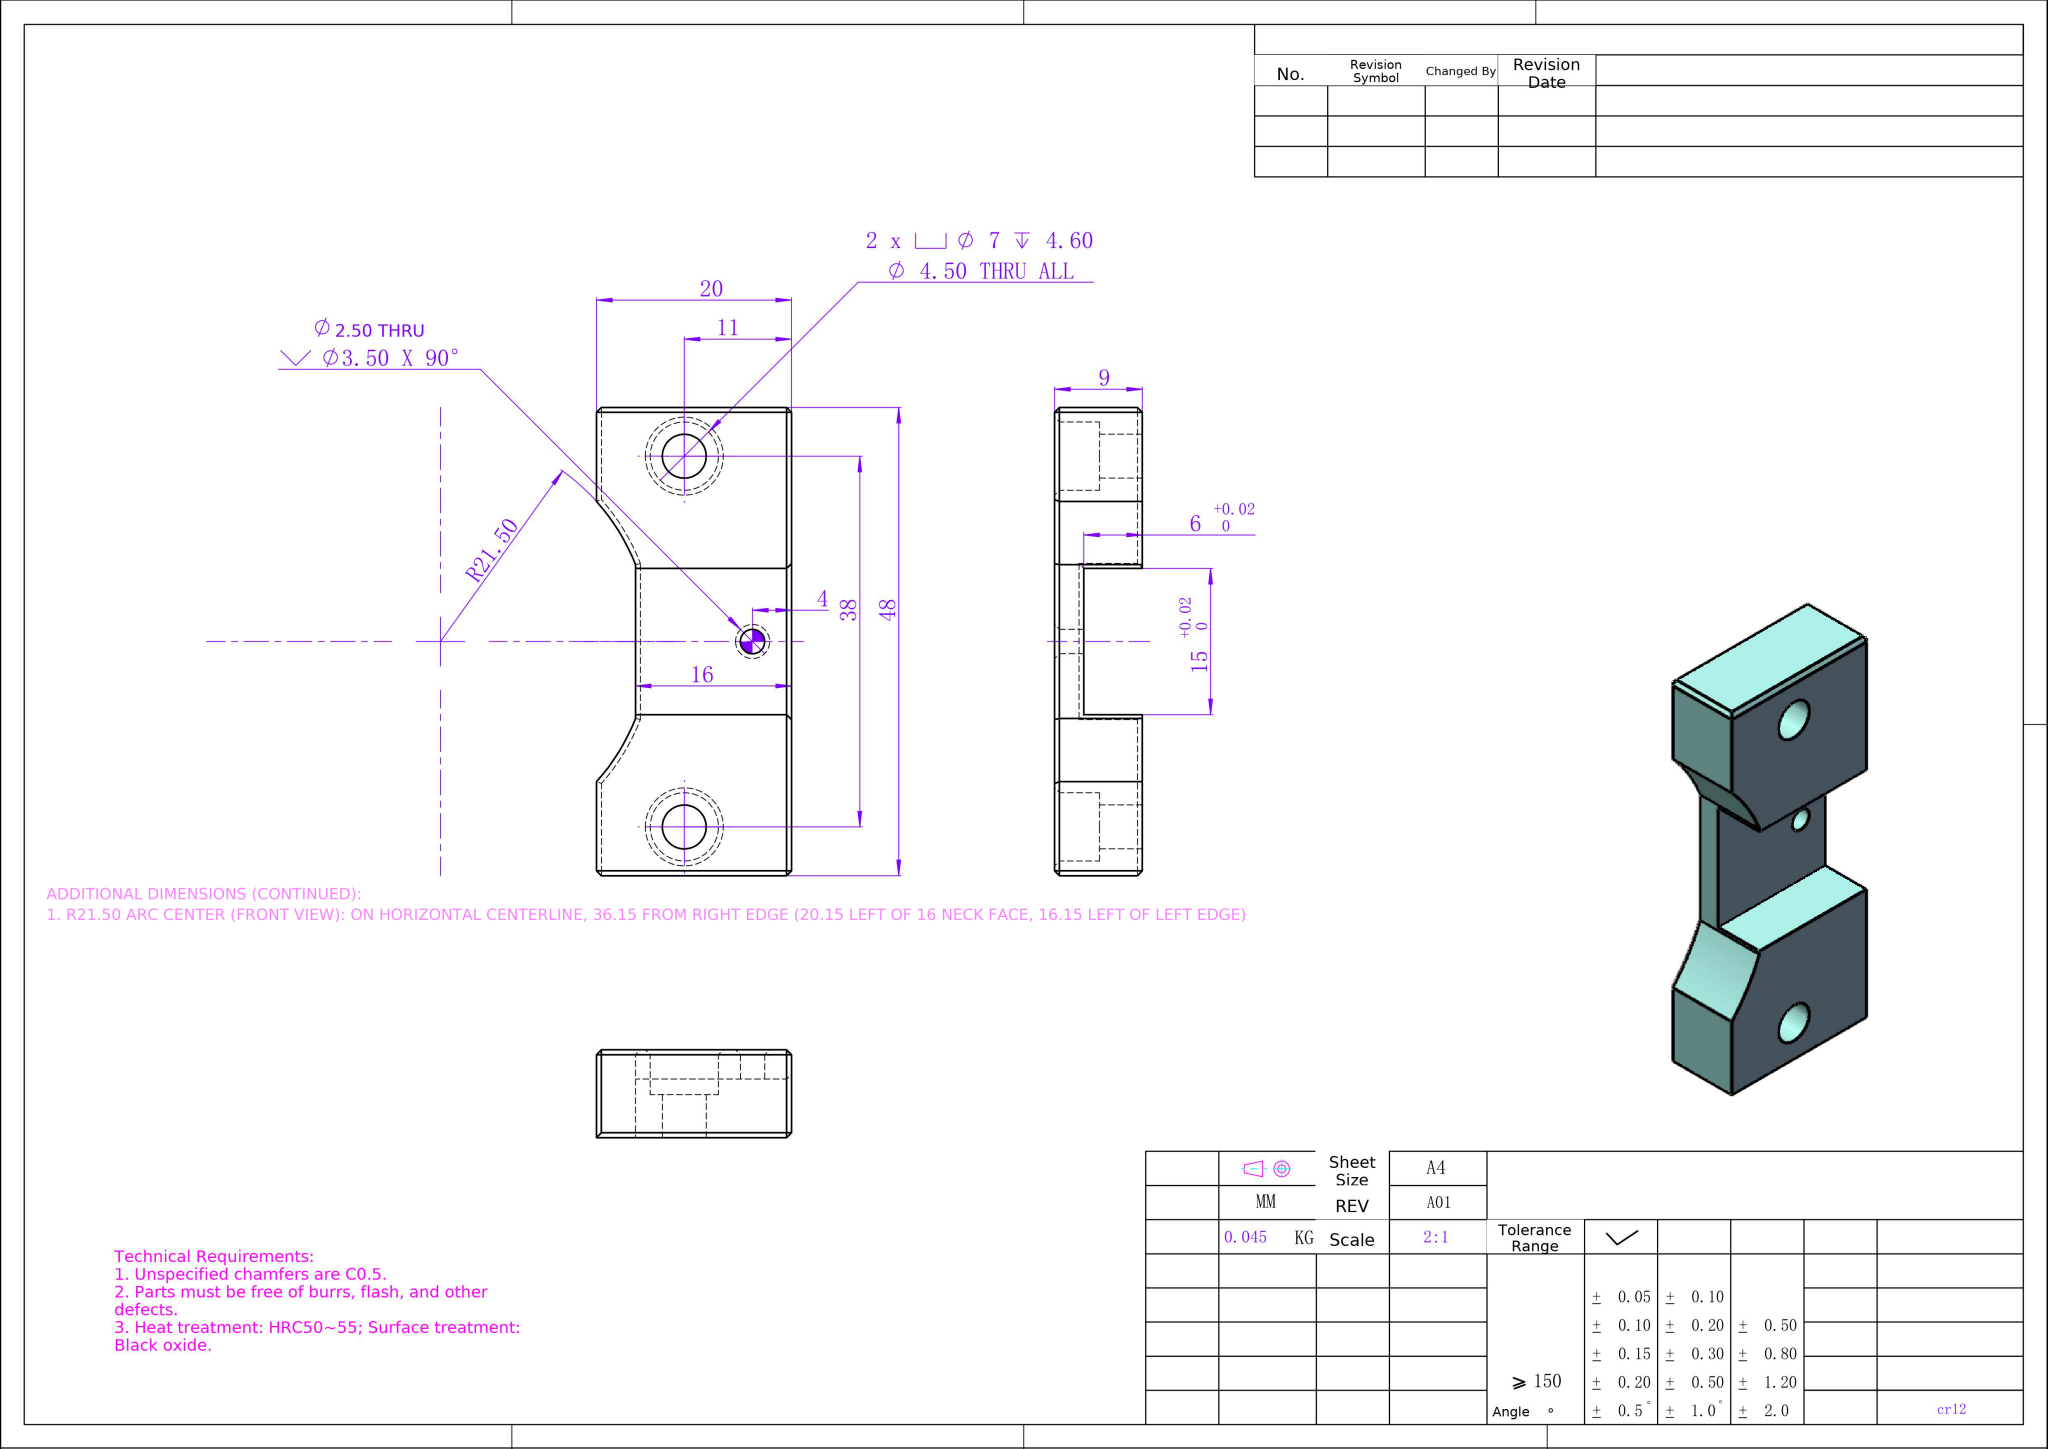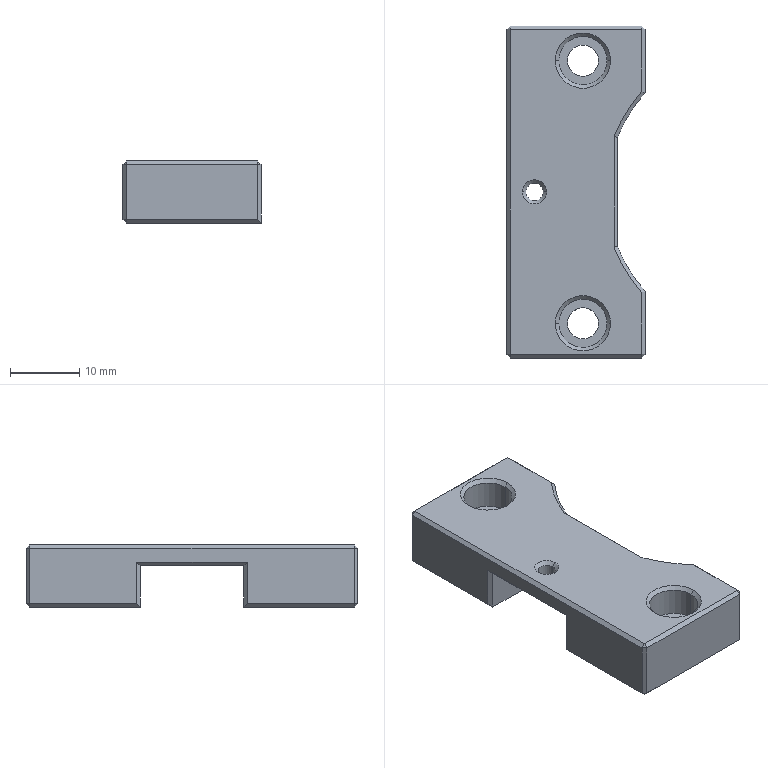Part | NX | mm | 1 solid | 57 faces | box 20 x 48 x 9 mm | volume 5819 mm3 | plane 37 | cylinder 12 | cone 8 | commonest cylinder face diameters 4.5 x4 7 x4 2.5 x2 43 x2